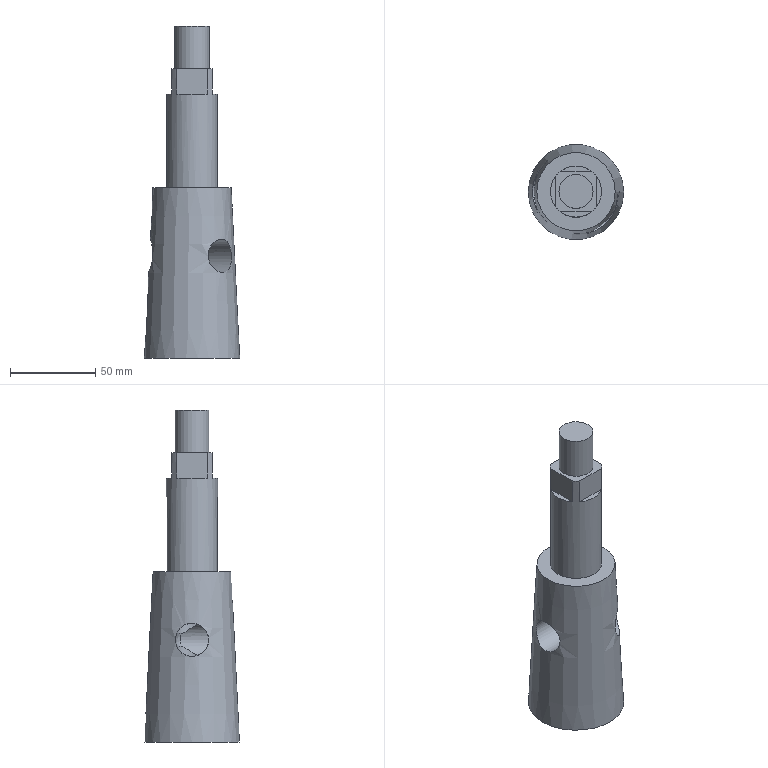Component | NX | VALVE_CORE | 1 solid | 21 faces | volume 228977 mm3 | plane 12 | cylinder 6 | cone 2 | sphere 1 | commonest cylinder face diameters 19.5 x2 18 x2 30 x1 20 x1